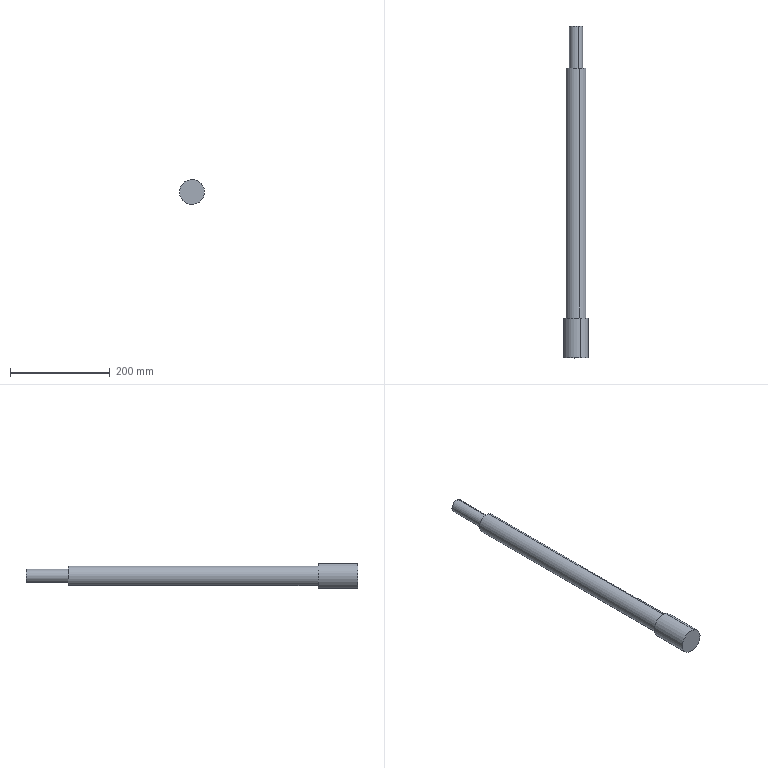Component | SolidWorks | BalanceCylinderLever-1 | 1 solid | 12 faces | box 50 x 665 x 50 mm | volume 832269 mm3 | cylinder 6 | plane 4 | cone 2 | commonest cylinder face diameters 26.5 x2 40 x2 50 x2
build123d program:
from build123d import *

# Parameters (mm, degrees)
SKETCH1_R           = 25
BOSS_EXTRUDE1_DEPTH = 80
SKETCH2_R           = 20
BOSS_EXTRUDE2_DEPTH = 500
SKETCH3_R           = 13.25
BOSS_EXTRUDE3_DEPTH = 85
CHAMFER1_SIZE       = 0.5


with BuildPart() as part:
    # Sketch1 → Boss-Extrude1 (new body)
    with BuildSketch(Plane.XY):
        Circle(SKETCH1_R)
    extrude(amount=-BOSS_EXTRUDE1_DEPTH)

    # Sketch2 → Boss-Extrude2 (add)
    with BuildSketch(Plane(origin=(0, 0, -80), x_dir=(-1, 0, 0), z_dir=(0, 0, -1))):
        with Locations(Location((0, 0, 0), (0, 0, 180))):
            Circle(SKETCH2_R)
    extrude(amount=BOSS_EXTRUDE2_DEPTH)

    # Sketch3 → Boss-Extrude3 (add)
    with BuildSketch(Plane(origin=(0, 0, -580), x_dir=(-1, 0, 0), z_dir=(0, 0, -1))):
        Circle(SKETCH3_R)
    extrude(amount=BOSS_EXTRUDE3_DEPTH)

    # Chamfer1
    chamfer1_edges = [part.edges().sort_by_distance(p)[0] for p in [
        (13.25, 0, -665),
    ]]
    chamfer(chamfer1_edges, length=CHAMFER1_SIZE)


solid = part.part

# Placed as in the assembly
solid = solid.moved(Location((-101.681, 510.897, 683.723), (90, 0, 0)))
STEP:
#1=COLOUR_RGB('',0.7922,0.8196,0.9333);
#2=FILL_AREA_STYLE_COLOUR('',#1);
#3=FILL_AREA_STYLE('',(#2));
#4=SURFACE_STYLE_FILL_AREA(#3);
#5=SURFACE_SIDE_STYLE('',(#4));
#6=SURFACE_STYLE_USAGE(.BOTH.,#5);
#7=PRESENTATION_STYLE_ASSIGNMENT((#6));
#8=CARTESIAN_POINT('',(-4.165,46.295,26.443));
#9=VERTEX_POINT('',#8);
#10=CARTESIAN_POINT('',(-3.842,46.295,27.393));
#11=VERTEX_POINT('',#10);
#12=CARTESIAN_POINT('',(-4.003,46.295,26.918));
#13=DIRECTION('',(0.,1.,-0.));
#14=DIRECTION('',(-0.322,0.,-0.9467));
#15=AXIS2_PLACEMENT_3D('',#12,#13,#14);
#16=CIRCLE('',#15,0.502);
#17=EDGE_CURVE('',#9,#11,#16,.T.);
#18=ORIENTED_EDGE('',*,*,#17,.F.);
#19=CARTESIAN_POINT('',(-4.171,46.275,26.424));
#20=VERTEX_POINT('',#19);
#21=CARTESIAN_POINT('',(-4.165,46.295,26.443));
#22=DIRECTION('',(-0.2277,-0.7071,-0.6694));
#23=VECTOR('',#22,39.37);
#24=LINE('',#21,#23);
#25=EDGE_CURVE('',#9,#20,#24,.T.);
#26=ORIENTED_EDGE('',*,*,#25,.T.);
#27=CARTESIAN_POINT('',(-3.835,46.275,27.412));
#28=VERTEX_POINT('',#27);
#29=CARTESIAN_POINT('',(-4.003,46.275,26.918));
#30=DIRECTION('',(-0.,-1.,0.));
#31=DIRECTION('',(-0.322,0.,-0.9467));
#32=AXIS2_PLACEMENT_3D('',#29,#30,#31);
#33=CIRCLE('',#32,0.5217);
#34=EDGE_CURVE('',#28,#20,#33,.T.);
#35=ORIENTED_EDGE('',*,*,#34,.F.);
#36=CARTESIAN_POINT('',(-3.842,46.295,27.393));
#37=DIRECTION('',(0.2277,-0.7071,0.6694));
#38=VECTOR('',#37,39.37);
#39=LINE('',#36,#38);
#40=EDGE_CURVE('',#11,#28,#39,.T.);
#41=ORIENTED_EDGE('',*,*,#40,.F.);
#42=EDGE_LOOP('',(#18,#26,#35,#41));
#43=FACE_OUTER_BOUND('',#42,.T.);
#44=CARTESIAN_POINT('',(-4.003,46.295,26.918));
#45=DIRECTION('',(-0.,-1.,0.));
#46=DIRECTION('',(0.322,0.,0.9467));
#47=AXIS2_PLACEMENT_3D('',#44,#45,#46);
#48=CONICAL_SURFACE('',#47,0.502,0.7854);
#49=ADVANCED_FACE('',(#43),#48,.T.);
#50=ORIENTED_EDGE('',*,*,#34,.T.);
#51=CARTESIAN_POINT('',(-4.171,42.949,26.424));
#52=VERTEX_POINT('',#51);
#53=CARTESIAN_POINT('',(-4.171,46.295,26.424));
#54=DIRECTION('',(-0.,-1.,0.));
#55=VECTOR('',#54,39.37);
#56=LINE('',#53,#55);
#57=EDGE_CURVE('',#20,#52,#56,.T.);
#58=ORIENTED_EDGE('',*,*,#57,.T.);
#59=CARTESIAN_POINT('',(-3.835,42.949,27.412));
#60=VERTEX_POINT('',#59);
#61=CARTESIAN_POINT('',(-4.003,42.949,26.918));
#62=DIRECTION('',(0.,1.,-0.));
#63=DIRECTION('',(-0.322,0.,-0.9467));
#64=AXIS2_PLACEMENT_3D('',#61,#62,#63);
#65=CIRCLE('',#64,0.5217);
#66=EDGE_CURVE('',#52,#60,#65,.T.);
#67=ORIENTED_EDGE('',*,*,#66,.T.);
#68=CARTESIAN_POINT('',(-3.835,46.295,27.412));
#69=DIRECTION('',(-0.,-1.,0.));
#70=VECTOR('',#69,39.37);
#71=LINE('',#68,#70);
#72=EDGE_CURVE('',#28,#60,#71,.T.);
#73=ORIENTED_EDGE('',*,*,#72,.F.);
#74=EDGE_LOOP('',(#50,#58,#67,#73));
#75=FACE_OUTER_BOUND('',#74,.T.);
#76=CARTESIAN_POINT('',(-4.003,46.295,26.918));
#77=DIRECTION('',(-0.,-1.,0.));
#78=DIRECTION('',(0.322,0.,0.9467));
#79=AXIS2_PLACEMENT_3D('',#76,#77,#78);
#80=CYLINDRICAL_SURFACE('',#79,0.5217);
#81=ADVANCED_FACE('',(#75),#80,.T.);
#82=CARTESIAN_POINT('',(-4.257,42.949,26.173));
#83=VERTEX_POINT('',#82);
#84=CARTESIAN_POINT('',(-3.75,42.949,27.664));
#85=VERTEX_POINT('',#84);
#86=CARTESIAN_POINT('',(-4.003,42.949,26.918));
#87=DIRECTION('',(0.,1.,-0.));
#88=DIRECTION('',(-0.322,0.,-0.9467));
#89=AXIS2_PLACEMENT_3D('',#86,#87,#88);
#90=CIRCLE('',#89,0.7874);
#91=EDGE_CURVE('',#83,#85,#90,.T.);
#92=ORIENTED_EDGE('',*,*,#91,.F.);
#93=CARTESIAN_POINT('',(-4.257,23.264,26.173));
#94=VERTEX_POINT('',#93);
#95=CARTESIAN_POINT('',(-4.257,42.949,26.173));
#96=DIRECTION('',(-0.,-1.,0.));
#97=VECTOR('',#96,39.37);
#98=LINE('',#95,#97);
#99=EDGE_CURVE('',#83,#94,#98,.T.);
#100=ORIENTED_EDGE('',*,*,#99,.T.);
#101=CARTESIAN_POINT('',(-3.75,23.264,27.664));
#102=VERTEX_POINT('',#101);
#103=CARTESIAN_POINT('',(-4.003,23.264,26.918));
#104=DIRECTION('',(0.,1.,-0.));
#105=DIRECTION('',(0.322,0.,0.9467));
#106=AXIS2_PLACEMENT_3D('',#103,#104,#105);
#107=CIRCLE('',#106,0.7874);
#108=EDGE_CURVE('',#94,#102,#107,.T.);
#109=ORIENTED_EDGE('',*,*,#108,.T.);
#110=CARTESIAN_POINT('',(-3.75,42.949,27.664));
#111=DIRECTION('',(-0.,-1.,0.));
#112=VECTOR('',#111,39.37);
#113=LINE('',#110,#112);
#114=EDGE_CURVE('',#85,#102,#113,.T.);
#115=ORIENTED_EDGE('',*,*,#114,.F.);
#116=EDGE_LOOP('',(#92,#100,#109,#115));
#117=FACE_OUTER_BOUND('',#116,.T.);
#118=CARTESIAN_POINT('',(-4.003,42.949,26.918));
#119=DIRECTION('',(-0.,-1.,0.));
#120=DIRECTION('',(0.322,0.,0.9467));
#121=AXIS2_PLACEMENT_3D('',#118,#119,#120);
#122=CYLINDRICAL_SURFACE('',#121,0.7874);
#123=ADVANCED_FACE('',(#117),#122,.T.);
#124=CARTESIAN_POINT('',(-3.686,23.264,27.85));
#125=VERTEX_POINT('',#124);
#126=CARTESIAN_POINT('',(-4.32,23.264,25.986));
#127=VERTEX_POINT('',#126);
#128=CARTESIAN_POINT('',(-4.003,23.264,26.918));
#129=DIRECTION('',(-0.,-1.,0.));
#130=DIRECTION('',(0.322,0.,0.9467));
#131=AXIS2_PLACEMENT_3D('',#128,#129,#130);
#132=CIRCLE('',#131,0.9843);
#133=EDGE_CURVE('',#125,#127,#132,.T.);
#134=ORIENTED_EDGE('',*,*,#133,.T.);
#135=CARTESIAN_POINT('',(-4.32,20.114,25.986));
#136=VERTEX_POINT('',#135);
#137=CARTESIAN_POINT('',(-4.32,23.264,25.986));
#138=DIRECTION('',(-0.,-1.,0.));
#139=VECTOR('',#138,39.37);
#140=LINE('',#137,#139);
#141=EDGE_CURVE('',#127,#136,#140,.T.);
#142=ORIENTED_EDGE('',*,*,#141,.T.);
#143=CARTESIAN_POINT('',(-3.686,20.114,27.85));
#144=VERTEX_POINT('',#143);
#145=CARTESIAN_POINT('',(-4.003,20.114,26.918));
#146=DIRECTION('',(-0.,-1.,0.));
#147=DIRECTION('',(0.322,0.,0.9467));
#148=AXIS2_PLACEMENT_3D('',#145,#146,#147);
#149=CIRCLE('',#148,0.9843);
#150=EDGE_CURVE('',#144,#136,#149,.T.);
#151=ORIENTED_EDGE('',*,*,#150,.F.);
#152=CARTESIAN_POINT('',(-3.686,23.264,27.85));
#153=DIRECTION('',(-0.,-1.,0.));
#154=VECTOR('',#153,39.37);
#155=LINE('',#152,#154);
#156=EDGE_CURVE('',#125,#144,#155,.T.);
#157=ORIENTED_EDGE('',*,*,#156,.F.);
#158=EDGE_LOOP('',(#134,#142,#151,#157));
#159=FACE_OUTER_BOUND('',#158,.T.);
#160=CARTESIAN_POINT('',(-4.003,23.264,26.918));
#161=DIRECTION('',(-0.,-1.,0.));
#162=DIRECTION('',(0.322,0.,0.9467));
#163=AXIS2_PLACEMENT_3D('',#160,#161,#162);
#164=CYLINDRICAL_SURFACE('',#163,0.9843);
#165=ADVANCED_FACE('',(#159),#164,.T.);
#166=CARTESIAN_POINT('',(-4.003,42.949,26.918));
#167=DIRECTION('',(0.,1.,-0.));
#168=DIRECTION('',(-0.322,0.,-0.9467));
#169=AXIS2_PLACEMENT_3D('',#166,#167,#168);
#170=CIRCLE('',#169,0.7874);
#171=EDGE_CURVE('',#85,#83,#170,.T.);
#172=ORIENTED_EDGE('',*,*,#171,.T.);
#173=ORIENTED_EDGE('',*,*,#91,.T.);
#174=EDGE_LOOP('',(#172,#173));
#175=FACE_OUTER_BOUND('',#174,.T.);
#176=CARTESIAN_POINT('',(-4.003,42.949,26.918));
#177=DIRECTION('',(0.,1.,-0.));
#178=DIRECTION('',(-0.322,0.,-0.9467));
#179=AXIS2_PLACEMENT_3D('',#176,#177,#178);
#180=CIRCLE('',#179,0.5217);
#181=EDGE_CURVE('',#60,#52,#180,.T.);
#182=ORIENTED_EDGE('',*,*,#181,.F.);
#183=ORIENTED_EDGE('',*,*,#66,.F.);
#184=EDGE_LOOP('',(#182,#183));
#185=FACE_BOUND('',#184,.T.);
#186=CARTESIAN_POINT('',(-4.003,42.949,26.918));
#187=DIRECTION('',(0.,1.,-0.));
#188=DIRECTION('',(-0.322,-0.,-0.9467));
#189=AXIS2_PLACEMENT_3D('',#186,#187,#188);
#190=PLANE('',#189);
#191=ADVANCED_FACE('',(#175,#185),#190,.T.);
#192=ORIENTED_EDGE('',*,*,#133,.F.);
#193=CARTESIAN_POINT('',(-4.003,23.264,26.918));
#194=DIRECTION('',(-0.,-1.,0.));
#195=DIRECTION('',(0.322,0.,0.9467));
#196=AXIS2_PLACEMENT_3D('',#193,#194,#195);
#197=CIRCLE('',#196,0.9843);
#198=EDGE_CURVE('',#127,#125,#197,.T.);
#199=ORIENTED_EDGE('',*,*,#198,.F.);
#200=EDGE_LOOP('',(#192,#199));
#201=FACE_OUTER_BOUND('',#200,.T.);
#202=CARTESIAN_POINT('',(-4.003,23.264,26.918));
#203=DIRECTION('',(0.,1.,-0.));
#204=DIRECTION('',(0.322,0.,0.9467));
#205=AXIS2_PLACEMENT_3D('',#202,#203,#204);
#206=CIRCLE('',#205,0.7874);
#207=EDGE_CURVE('',#102,#94,#206,.T.);
#208=ORIENTED_EDGE('',*,*,#207,.F.);
#209=ORIENTED_EDGE('',*,*,#108,.F.);
#210=EDGE_LOOP('',(#208,#209));
#211=FACE_BOUND('',#210,.T.);
#212=CARTESIAN_POINT('',(-4.003,23.264,26.918));
#213=DIRECTION('',(-0.,-1.,0.));
#214=DIRECTION('',(0.322,0.,0.9467));
#215=AXIS2_PLACEMENT_3D('',#212,#213,#214);
#216=PLANE('',#215);
#217=ADVANCED_FACE('',(#201,#211),#216,.F.);
#218=ORIENTED_EDGE('',*,*,#141,.F.);
#219=ORIENTED_EDGE('',*,*,#198,.T.);
#220=ORIENTED_EDGE('',*,*,#156,.T.);
#221=CARTESIAN_POINT('',(-4.003,20.114,26.918));
#222=DIRECTION('',(-0.,-1.,0.));
#223=DIRECTION('',(0.322,0.,0.9467));
#224=AXIS2_PLACEMENT_3D('',#221,#222,#223);
#225=CIRCLE('',#224,0.9843);
#226=EDGE_CURVE('',#136,#144,#225,.T.);
#227=ORIENTED_EDGE('',*,*,#226,.F.);
#228=EDGE_LOOP('',(#218,#219,#220,#227));
#229=FACE_OUTER_BOUND('',#228,.T.);
#230=CARTESIAN_POINT('',(-4.003,23.264,26.918));
#231=DIRECTION('',(-0.,-1.,0.));
#232=DIRECTION('',(0.322,0.,0.9467));
#233=AXIS2_PLACEMENT_3D('',#230,#231,#232);
#234=CYLINDRICAL_SURFACE('',#233,0.9843);
#235=ADVANCED_FACE('',(#229),#234,.T.);
#236=ORIENTED_EDGE('',*,*,#150,.T.);
#237=ORIENTED_EDGE('',*,*,#226,.T.);
#238=EDGE_LOOP('',(#236,#237));
#239=FACE_OUTER_BOUND('',#238,.T.);
#240=CARTESIAN_POINT('',(-4.003,20.114,26.918));
#241=DIRECTION('',(-0.,-1.,0.));
#242=DIRECTION('',(0.322,0.,0.9467));
#243=AXIS2_PLACEMENT_3D('',#240,#241,#242);
#244=PLANE('',#243);
#245=ADVANCED_FACE('',(#239),#244,.T.);
#246=ORIENTED_EDGE('',*,*,#99,.F.);
#247=ORIENTED_EDGE('',*,*,#171,.F.);
#248=ORIENTED_EDGE('',*,*,#114,.T.);
#249=ORIENTED_EDGE('',*,*,#207,.T.);
#250=EDGE_LOOP('',(#246,#247,#248,#249));
#251=FACE_OUTER_BOUND('',#250,.T.);
#252=CARTESIAN_POINT('',(-4.003,42.949,26.918));
#253=DIRECTION('',(-0.,-1.,0.));
#254=DIRECTION('',(0.322,0.,0.9467));
#255=AXIS2_PLACEMENT_3D('',#252,#253,#254);
#256=CYLINDRICAL_SURFACE('',#255,0.7874);
#257=ADVANCED_FACE('',(#251),#256,.T.);
#258=ORIENTED_EDGE('',*,*,#57,.F.);
#259=CARTESIAN_POINT('',(-4.003,46.275,26.918));
#260=DIRECTION('',(-0.,-1.,0.));
#261=DIRECTION('',(-0.322,0.,-0.9467));
#262=AXIS2_PLACEMENT_3D('',#259,#260,#261);
#263=CIRCLE('',#262,0.5217);
#264=EDGE_CURVE('',#20,#28,#263,.T.);
#265=ORIENTED_EDGE('',*,*,#264,.T.);
#266=ORIENTED_EDGE('',*,*,#72,.T.);
#267=ORIENTED_EDGE('',*,*,#181,.T.);
#268=EDGE_LOOP('',(#258,#265,#266,#267));
#269=FACE_OUTER_BOUND('',#268,.T.);
#270=CARTESIAN_POINT('',(-4.003,46.295,26.918));
#271=DIRECTION('',(-0.,-1.,0.));
#272=DIRECTION('',(0.322,0.,0.9467));
#273=AXIS2_PLACEMENT_3D('',#270,#271,#272);
#274=CYLINDRICAL_SURFACE('',#273,0.5217);
#275=ADVANCED_FACE('',(#269),#274,.T.);
#276=CARTESIAN_POINT('',(-4.003,46.295,26.918));
#277=DIRECTION('',(0.,1.,-0.));
#278=DIRECTION('',(-0.322,0.,-0.9467));
#279=AXIS2_PLACEMENT_3D('',#276,#277,#278);
#280=CIRCLE('',#279,0.502);
#281=EDGE_CURVE('',#11,#9,#280,.T.);
#282=ORIENTED_EDGE('',*,*,#281,.T.);
#283=ORIENTED_EDGE('',*,*,#17,.T.);
#284=EDGE_LOOP('',(#282,#283));
#285=FACE_OUTER_BOUND('',#284,.T.);
#286=CARTESIAN_POINT('',(-4.003,46.295,26.918));
#287=DIRECTION('',(0.,1.,-0.));
#288=DIRECTION('',(-0.322,-0.,-0.9467));
#289=AXIS2_PLACEMENT_3D('',#286,#287,#288);
#290=PLANE('',#289);
#291=ADVANCED_FACE('',(#285),#290,.T.);
#292=ORIENTED_EDGE('',*,*,#25,.F.);
#293=ORIENTED_EDGE('',*,*,#281,.F.);
#294=ORIENTED_EDGE('',*,*,#40,.T.);
#295=ORIENTED_EDGE('',*,*,#264,.F.);
#296=EDGE_LOOP('',(#292,#293,#294,#295));
#297=FACE_OUTER_BOUND('',#296,.T.);
#298=CARTESIAN_POINT('',(-4.003,46.295,26.918));
#299=DIRECTION('',(-0.,-1.,0.));
#300=DIRECTION('',(0.322,0.,0.9467));
#301=AXIS2_PLACEMENT_3D('',#298,#299,#300);
#302=CONICAL_SURFACE('',#301,0.502,0.7854);
#303=ADVANCED_FACE('',(#297),#302,.T.);
#304=CLOSED_SHELL('',(#49,#81,#123,#165,#191,#217,#235,#245,#257,#275,#291,#303));
#305=MANIFOLD_SOLID_BREP('',#304);
#306=STYLED_ITEM('',(#7),#305);
#307=(LENGTH_UNIT()NAMED_UNIT(*)SI_UNIT($,.METRE.));
#308=LENGTH_MEASURE_WITH_UNIT(LENGTH_MEASURE(0.0254),#307);
#309=DIMENSIONAL_EXPONENTS(1.,0.,0.,0.,0.,0.,0.);
#310=(CONVERSION_BASED_UNIT('',#308)LENGTH_UNIT()NAMED_UNIT(#309));
#311=UNCERTAINTY_MEASURE_WITH_UNIT(LENGTH_MEASURE(0.00001),#310,'','');
#312=(NAMED_UNIT(*)PLANE_ANGLE_UNIT()SI_UNIT($,.RADIAN.));
#313=(NAMED_UNIT(*)SI_UNIT($,.STERADIAN.)SOLID_ANGLE_UNIT());
#314=(GEOMETRIC_REPRESENTATION_CONTEXT(3)GLOBAL_UNCERTAINTY_ASSIGNED_CONTEXT((#311))GLOBAL_UNIT_ASSIGNED_CONTEXT((#310,#312,#313))REPRESENTATION_CONTEXT('',''));
#315=MECHANICAL_DESIGN_GEOMETRIC_PRESENTATION_REPRESENTATION('',(#306),#314);
#316=CARTESIAN_POINT('',(0.,0.,0.));
#317=DIRECTION('',(0.,0.,1.));
#318=DIRECTION('',(1.,0.,0.));
#319=AXIS2_PLACEMENT_3D('',#316,#317,#318);
#320=(LENGTH_UNIT()NAMED_UNIT(*)SI_UNIT($,.METRE.));
#321=LENGTH_MEASURE_WITH_UNIT(LENGTH_MEASURE(0.0254),#320);
#322=DIMENSIONAL_EXPONENTS(1.,0.,0.,0.,0.,0.,0.);
#323=(CONVERSION_BASED_UNIT('',#321)LENGTH_UNIT()NAMED_UNIT(#322));
#324=UNCERTAINTY_MEASURE_WITH_UNIT(LENGTH_MEASURE(0.00001),#323,'','');
#325=(NAMED_UNIT(*)PLANE_ANGLE_UNIT()SI_UNIT($,.RADIAN.));
#326=(NAMED_UNIT(*)SI_UNIT($,.STERADIAN.)SOLID_ANGLE_UNIT());
#327=(GEOMETRIC_REPRESENTATION_CONTEXT(3)GLOBAL_UNCERTAINTY_ASSIGNED_CONTEXT((#324))GLOBAL_UNIT_ASSIGNED_CONTEXT((#323,#325,#326))REPRESENTATION_CONTEXT('',''));
#328=ADVANCED_BREP_SHAPE_REPRESENTATION('',(#305,#319),#327);
#329=PRESENTATION_LAYER_ASSIGNMENT('','',(#306));